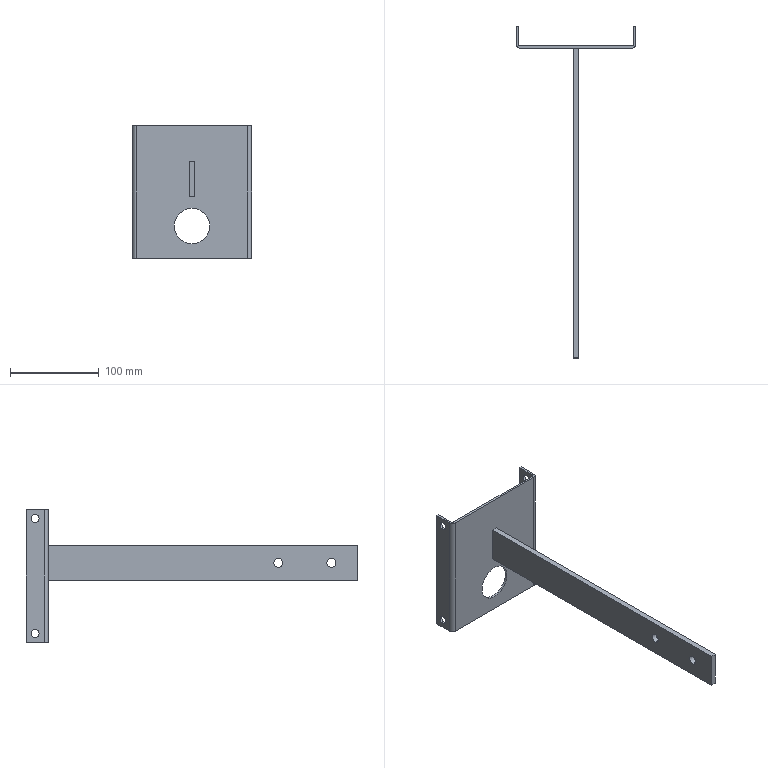Component | SolidWorks | SeedBoxBracket-1 | 1 solid | 33 faces | box 135 x 375 x 150 mm | volume 145734 mm3 | cylinder 18 | plane 15 | commonest cylinder face diameters 9 x10 10 x4 40 x2 4 x2
build123d program:
from build123d import *

# Parameters (mm, degrees)
EXTRUDE_THIN1_DEPTH = 75
SKETCH2_R           = 4.5
CUT_EXTRUDE1_DEPTH  = 157.445
SKETCH3_W           = 6
SKETCH3_H           = 40
BOSS_EXTRUDE1_DEPTH = 350
SKETCH4_R           = 5
CUT_EXTRUDE2_DEPTH  = 400
SKETCH5_R           = 20
CUT_EXTRUDE3_DEPTH  = 10


with BuildPart() as part:
    # Sketch1 → Extrude-Thin1 (new, symmetric)
    with BuildSketch(Plane.XY):
        with BuildLine():
            Line((-67.5, 25), (-67.5, 4.5))
            ThreePointArc((-67.5, 4.5), (-66.182, 1.318), (-63, 0))
            Line((-63, 0), (63, 0))
            ThreePointArc((63, 0), (66.182, 1.318), (67.5, 4.5))
            Line((67.5, 4.5), (67.5, 25))
            Line((67.5, 25), (65, 25))
            Line((65, 25), (65, 4.5))
            ThreePointArc((65, 4.5), (64.414, 3.086), (63, 2.5))
            Line((63, 2.5), (-63, 2.5))
            ThreePointArc((-63, 2.5), (-64.414, 3.086), (-65, 4.5))
            Line((-65, 4.5), (-65, 25))
            Line((-65, 25), (-67.5, 25))
        make_face()
    extrude(amount=EXTRUDE_THIN1_DEPTH, both=True)

    # Sketch2 → Cut-Extrude1 (cut, through all)
    with BuildSketch(Plane.ZY.offset(67.5)):
        with Locations(Location((-65, 14.75, 0), (0, 0, 270))):
            Circle(SKETCH2_R)
        with Locations(Location((65, 14.75, 0), (0, 0, 270))):
            Circle(SKETCH2_R)
    extrude(amount=-CUT_EXTRUDE1_DEPTH, mode=Mode.SUBTRACT)

    # Sketch3 → Boss-Extrude1 (add)
    with BuildSketch(Plane.XZ):
        with Locations((0, -15)):
            Rectangle(SKETCH3_W, SKETCH3_H)
    extrude(amount=BOSS_EXTRUDE1_DEPTH)

    # Sketch4 → Cut-Extrude2 (cut)
    with BuildSketch(Plane.ZY.offset(3)):
        with Locations((-15, -320)):
            Circle(SKETCH4_R)
        with Locations((-15, -260)):
            Circle(SKETCH4_R)
    extrude(amount=-CUT_EXTRUDE2_DEPTH, mode=Mode.SUBTRACT)

    # Sketch5 → Cut-Extrude3 (cut)
    with BuildSketch(Plane(origin=(0, 2.5, 0), x_dir=(1, 0, 0), z_dir=(0, 1, 0))):
        with Locations(Location((0, -38.536, 0), (0, 0, 270))):
            Circle(SKETCH5_R)
    extrude(amount=-CUT_EXTRUDE3_DEPTH, mode=Mode.SUBTRACT)


solid = part.part

# Placed as in the assembly
solid = solid.moved(Location((-5.5, 260, -327.5), (-180, 0, 180)))
STEP:
#1=CARTESIAN_POINT('',(-0.2165,10.236,-13.623));
#2=VERTEX_POINT('',#1);
#3=CARTESIAN_POINT('',(-0.2165,10.236,-15.198));
#4=VERTEX_POINT('',#3);
#5=CARTESIAN_POINT('',(-0.2165,10.236,-14.411));
#6=DIRECTION('',(-0.,1.,0.));
#7=DIRECTION('',(-0.,0.,-1.));
#8=AXIS2_PLACEMENT_3D('',#5,#6,#7);
#9=CIRCLE('',#8,0.7874);
#10=EDGE_CURVE('',#2,#4,#9,.T.);
#11=ORIENTED_EDGE('',*,*,#10,.F.);
#12=CARTESIAN_POINT('',(-0.2165,10.335,-13.623));
#13=VERTEX_POINT('',#12);
#14=CARTESIAN_POINT('',(-0.2165,9.941,-13.623));
#15=DIRECTION('',(-0.,1.,0.));
#16=VECTOR('',#15,39.37);
#17=LINE('',#14,#16);
#18=EDGE_CURVE('',#2,#13,#17,.T.);
#19=ORIENTED_EDGE('',*,*,#18,.T.);
#20=CARTESIAN_POINT('',(-0.2165,10.335,-15.198));
#21=VERTEX_POINT('',#20);
#22=CARTESIAN_POINT('',(-0.2165,10.335,-14.411));
#23=DIRECTION('',(-0.,1.,0.));
#24=DIRECTION('',(-0.,0.,-1.));
#25=AXIS2_PLACEMENT_3D('',#22,#23,#24);
#26=CIRCLE('',#25,0.7874);
#27=EDGE_CURVE('',#13,#21,#26,.T.);
#28=ORIENTED_EDGE('',*,*,#27,.T.);
#29=CARTESIAN_POINT('',(-0.2165,9.941,-15.198));
#30=DIRECTION('',(-0.,1.,0.));
#31=VECTOR('',#30,39.37);
#32=LINE('',#29,#31);
#33=EDGE_CURVE('',#4,#21,#32,.T.);
#34=ORIENTED_EDGE('',*,*,#33,.F.);
#35=EDGE_LOOP('',(#11,#19,#28,#34));
#36=FACE_OUTER_BOUND('',#35,.T.);
#37=CARTESIAN_POINT('',(-0.2165,9.941,-14.411));
#38=DIRECTION('',(-0.,1.,0.));
#39=DIRECTION('',(-0.,0.,-1.));
#40=AXIS2_PLACEMENT_3D('',#37,#38,#39);
#41=CYLINDRICAL_SURFACE('',#40,0.7874);
#42=ADVANCED_FACE('',(#36),#41,.F.);
#43=CARTESIAN_POINT('',(-0.3346,0.,-12.106));
#44=VERTEX_POINT('',#43);
#45=CARTESIAN_POINT('',(-0.3346,0.,-12.5));
#46=VERTEX_POINT('',#45);
#47=CARTESIAN_POINT('',(-0.3346,0.,-12.303));
#48=DIRECTION('',(1.,0.,-0.));
#49=DIRECTION('',(0.,0.,-1.));
#50=AXIS2_PLACEMENT_3D('',#47,#48,#49);
#51=CIRCLE('',#50,0.1969);
#52=EDGE_CURVE('',#44,#46,#51,.T.);
#53=ORIENTED_EDGE('',*,*,#52,.F.);
#54=CARTESIAN_POINT('',(-0.09843,0.,-12.106));
#55=VERTEX_POINT('',#54);
#56=CARTESIAN_POINT('',(-15.846,0.,-12.106));
#57=DIRECTION('',(1.,0.,-0.));
#58=VECTOR('',#57,39.37);
#59=LINE('',#56,#58);
#60=EDGE_CURVE('',#44,#55,#59,.T.);
#61=ORIENTED_EDGE('',*,*,#60,.T.);
#62=CARTESIAN_POINT('',(-0.09843,0.,-12.5));
#63=VERTEX_POINT('',#62);
#64=CARTESIAN_POINT('',(-0.09843,0.,-12.303));
#65=DIRECTION('',(1.,0.,-0.));
#66=DIRECTION('',(-0.,0.,-1.));
#67=AXIS2_PLACEMENT_3D('',#64,#65,#66);
#68=CIRCLE('',#67,0.1969);
#69=EDGE_CURVE('',#55,#63,#68,.T.);
#70=ORIENTED_EDGE('',*,*,#69,.T.);
#71=CARTESIAN_POINT('',(-15.846,0.,-12.5));
#72=DIRECTION('',(1.,0.,-0.));
#73=VECTOR('',#72,39.37);
#74=LINE('',#71,#73);
#75=EDGE_CURVE('',#46,#63,#74,.T.);
#76=ORIENTED_EDGE('',*,*,#75,.F.);
#77=EDGE_LOOP('',(#53,#61,#70,#76));
#78=FACE_OUTER_BOUND('',#77,.T.);
#79=CARTESIAN_POINT('',(-15.846,0.,-12.303));
#80=DIRECTION('',(1.,0.,-0.));
#81=DIRECTION('',(0.,0.,-1.));
#82=AXIS2_PLACEMENT_3D('',#79,#80,#81);
#83=CYLINDRICAL_SURFACE('',#82,0.1969);
#84=ADVANCED_FACE('',(#78),#83,.F.);
#85=CARTESIAN_POINT('',(-0.3346,-2.362,-12.106));
#86=VERTEX_POINT('',#85);
#87=CARTESIAN_POINT('',(-0.3346,-2.362,-12.5));
#88=VERTEX_POINT('',#87);
#89=CARTESIAN_POINT('',(-0.3346,-2.362,-12.303));
#90=DIRECTION('',(1.,0.,-0.));
#91=DIRECTION('',(0.,0.,-1.));
#92=AXIS2_PLACEMENT_3D('',#89,#90,#91);
#93=CIRCLE('',#92,0.1969);
#94=EDGE_CURVE('',#86,#88,#93,.T.);
#95=ORIENTED_EDGE('',*,*,#94,.F.);
#96=CARTESIAN_POINT('',(-0.09843,-2.362,-12.106));
#97=VERTEX_POINT('',#96);
#98=CARTESIAN_POINT('',(-15.846,-2.362,-12.106));
#99=DIRECTION('',(1.,0.,-0.));
#100=VECTOR('',#99,39.37);
#101=LINE('',#98,#100);
#102=EDGE_CURVE('',#86,#97,#101,.T.);
#103=ORIENTED_EDGE('',*,*,#102,.T.);
#104=CARTESIAN_POINT('',(-0.09843,-2.362,-12.5));
#105=VERTEX_POINT('',#104);
#106=CARTESIAN_POINT('',(-0.09843,-2.362,-12.303));
#107=DIRECTION('',(1.,0.,-0.));
#108=DIRECTION('',(-0.,0.,-1.));
#109=AXIS2_PLACEMENT_3D('',#106,#107,#108);
#110=CIRCLE('',#109,0.1969);
#111=EDGE_CURVE('',#97,#105,#110,.T.);
#112=ORIENTED_EDGE('',*,*,#111,.T.);
#113=CARTESIAN_POINT('',(-15.846,-2.362,-12.5));
#114=DIRECTION('',(1.,0.,-0.));
#115=VECTOR('',#114,39.37);
#116=LINE('',#113,#115);
#117=EDGE_CURVE('',#88,#105,#116,.T.);
#118=ORIENTED_EDGE('',*,*,#117,.F.);
#119=EDGE_LOOP('',(#95,#103,#112,#118));
#120=FACE_OUTER_BOUND('',#119,.T.);
#121=CARTESIAN_POINT('',(-15.846,-2.362,-12.303));
#122=DIRECTION('',(1.,0.,-0.));
#123=DIRECTION('',(0.,0.,-1.));
#124=AXIS2_PLACEMENT_3D('',#121,#122,#123);
#125=CYLINDRICAL_SURFACE('',#124,0.1969);
#126=ADVANCED_FACE('',(#120),#125,.F.);
#127=CARTESIAN_POINT('',(-2.874,10.994,-15.453));
#128=VERTEX_POINT('',#127);
#129=CARTESIAN_POINT('',(-2.874,10.64,-15.453));
#130=VERTEX_POINT('',#129);
#131=CARTESIAN_POINT('',(-2.874,10.817,-15.453));
#132=DIRECTION('',(1.,-0.,-0.));
#133=DIRECTION('',(0.,-1.,0.));
#134=AXIS2_PLACEMENT_3D('',#131,#132,#133);
#135=CIRCLE('',#134,0.1772);
#136=EDGE_CURVE('',#128,#130,#135,.T.);
#137=ORIENTED_EDGE('',*,*,#136,.F.);
#138=CARTESIAN_POINT('',(-2.776,10.994,-15.453));
#139=VERTEX_POINT('',#138);
#140=CARTESIAN_POINT('',(-2.874,10.994,-15.453));
#141=DIRECTION('',(1.,-0.,-0.));
#142=VECTOR('',#141,39.37);
#143=LINE('',#140,#142);
#144=EDGE_CURVE('',#128,#139,#143,.T.);
#145=ORIENTED_EDGE('',*,*,#144,.T.);
#146=CARTESIAN_POINT('',(-2.776,10.64,-15.453));
#147=VERTEX_POINT('',#146);
#148=CARTESIAN_POINT('',(-2.776,10.817,-15.453));
#149=DIRECTION('',(1.,0.,-0.));
#150=DIRECTION('',(0.,0.,-1.));
#151=AXIS2_PLACEMENT_3D('',#148,#149,#150);
#152=CIRCLE('',#151,0.1772);
#153=EDGE_CURVE('',#139,#147,#152,.T.);
#154=ORIENTED_EDGE('',*,*,#153,.T.);
#155=CARTESIAN_POINT('',(-2.874,10.64,-15.453));
#156=DIRECTION('',(1.,-0.,-0.));
#157=VECTOR('',#156,39.37);
#158=LINE('',#155,#157);
#159=EDGE_CURVE('',#130,#147,#158,.T.);
#160=ORIENTED_EDGE('',*,*,#159,.F.);
#161=EDGE_LOOP('',(#137,#145,#154,#160));
#162=FACE_OUTER_BOUND('',#161,.T.);
#163=CARTESIAN_POINT('',(-2.874,10.817,-15.453));
#164=DIRECTION('',(1.,-0.,-0.));
#165=DIRECTION('',(0.,-1.,0.));
#166=AXIS2_PLACEMENT_3D('',#163,#164,#165);
#167=CYLINDRICAL_SURFACE('',#166,0.1772);
#168=ADVANCED_FACE('',(#162),#167,.F.);
#169=CARTESIAN_POINT('',(2.343,10.64,-15.453));
#170=VERTEX_POINT('',#169);
#171=CARTESIAN_POINT('',(2.343,10.994,-15.453));
#172=VERTEX_POINT('',#171);
#173=CARTESIAN_POINT('',(2.343,10.817,-15.453));
#174=DIRECTION('',(-1.,-0.,0.));
#175=DIRECTION('',(0.,0.,1.));
#176=AXIS2_PLACEMENT_3D('',#173,#174,#175);
#177=CIRCLE('',#176,0.1772);
#178=EDGE_CURVE('',#170,#172,#177,.T.);
#179=ORIENTED_EDGE('',*,*,#178,.T.);
#180=CARTESIAN_POINT('',(2.441,10.994,-15.453));
#181=VERTEX_POINT('',#180);
#182=CARTESIAN_POINT('',(-2.874,10.994,-15.453));
#183=DIRECTION('',(1.,-0.,-0.));
#184=VECTOR('',#183,39.37);
#185=LINE('',#182,#184);
#186=EDGE_CURVE('',#172,#181,#185,.T.);
#187=ORIENTED_EDGE('',*,*,#186,.T.);
#188=CARTESIAN_POINT('',(2.441,10.64,-15.453));
#189=VERTEX_POINT('',#188);
#190=CARTESIAN_POINT('',(2.441,10.817,-15.453));
#191=DIRECTION('',(1.,-0.,-0.));
#192=DIRECTION('',(0.,-1.,0.));
#193=AXIS2_PLACEMENT_3D('',#190,#191,#192);
#194=CIRCLE('',#193,0.1772);
#195=EDGE_CURVE('',#181,#189,#194,.T.);
#196=ORIENTED_EDGE('',*,*,#195,.T.);
#197=CARTESIAN_POINT('',(-2.874,10.64,-15.453));
#198=DIRECTION('',(1.,-0.,-0.));
#199=VECTOR('',#198,39.37);
#200=LINE('',#197,#199);
#201=EDGE_CURVE('',#170,#189,#200,.T.);
#202=ORIENTED_EDGE('',*,*,#201,.F.);
#203=EDGE_LOOP('',(#179,#187,#196,#202));
#204=FACE_OUTER_BOUND('',#203,.T.);
#205=CARTESIAN_POINT('',(-2.874,10.817,-15.453));
#206=DIRECTION('',(1.,-0.,-0.));
#207=DIRECTION('',(0.,-1.,0.));
#208=AXIS2_PLACEMENT_3D('',#205,#206,#207);
#209=CYLINDRICAL_SURFACE('',#208,0.1772);
#210=ADVANCED_FACE('',(#204),#209,.F.);
#211=CARTESIAN_POINT('',(-2.874,10.994,-10.335));
#212=VERTEX_POINT('',#211);
#213=CARTESIAN_POINT('',(-2.874,10.64,-10.335));
#214=VERTEX_POINT('',#213);
#215=CARTESIAN_POINT('',(-2.874,10.817,-10.335));
#216=DIRECTION('',(1.,-0.,-0.));
#217=DIRECTION('',(0.,-1.,0.));
#218=AXIS2_PLACEMENT_3D('',#215,#216,#217);
#219=CIRCLE('',#218,0.1772);
#220=EDGE_CURVE('',#212,#214,#219,.T.);
#221=ORIENTED_EDGE('',*,*,#220,.F.);
#222=CARTESIAN_POINT('',(-2.776,10.994,-10.335));
#223=VERTEX_POINT('',#222);
#224=CARTESIAN_POINT('',(-2.874,10.994,-10.335));
#225=DIRECTION('',(1.,-0.,-0.));
#226=VECTOR('',#225,39.37);
#227=LINE('',#224,#226);
#228=EDGE_CURVE('',#212,#223,#227,.T.);
#229=ORIENTED_EDGE('',*,*,#228,.T.);
#230=CARTESIAN_POINT('',(-2.776,10.64,-10.335));
#231=VERTEX_POINT('',#230);
#232=CARTESIAN_POINT('',(-2.776,10.817,-10.335));
#233=DIRECTION('',(1.,0.,-0.));
#234=DIRECTION('',(0.,0.,-1.));
#235=AXIS2_PLACEMENT_3D('',#232,#233,#234);
#236=CIRCLE('',#235,0.1772);
#237=EDGE_CURVE('',#223,#231,#236,.T.);
#238=ORIENTED_EDGE('',*,*,#237,.T.);
#239=CARTESIAN_POINT('',(-2.874,10.64,-10.335));
#240=DIRECTION('',(1.,-0.,-0.));
#241=VECTOR('',#240,39.37);
#242=LINE('',#239,#241);
#243=EDGE_CURVE('',#214,#231,#242,.T.);
#244=ORIENTED_EDGE('',*,*,#243,.F.);
#245=EDGE_LOOP('',(#221,#229,#238,#244));
#246=FACE_OUTER_BOUND('',#245,.T.);
#247=CARTESIAN_POINT('',(-2.874,10.817,-10.335));
#248=DIRECTION('',(1.,-0.,-0.));
#249=DIRECTION('',(0.,-1.,0.));
#250=AXIS2_PLACEMENT_3D('',#247,#248,#249);
#251=CYLINDRICAL_SURFACE('',#250,0.1772);
#252=ADVANCED_FACE('',(#246),#251,.F.);
#253=CARTESIAN_POINT('',(2.343,10.64,-10.335));
#254=VERTEX_POINT('',#253);
#255=CARTESIAN_POINT('',(2.343,10.994,-10.335));
#256=VERTEX_POINT('',#255);
#257=CARTESIAN_POINT('',(2.343,10.817,-10.335));
#258=DIRECTION('',(-1.,-0.,0.));
#259=DIRECTION('',(0.,0.,1.));
#260=AXIS2_PLACEMENT_3D('',#257,#258,#259);
#261=CIRCLE('',#260,0.1772);
#262=EDGE_CURVE('',#254,#256,#261,.T.);
#263=ORIENTED_EDGE('',*,*,#262,.T.);
#264=CARTESIAN_POINT('',(2.441,10.994,-10.335));
#265=VERTEX_POINT('',#264);
#266=CARTESIAN_POINT('',(-2.874,10.994,-10.335));
#267=DIRECTION('',(1.,-0.,-0.));
#268=VECTOR('',#267,39.37);
#269=LINE('',#266,#268);
#270=EDGE_CURVE('',#256,#265,#269,.T.);
#271=ORIENTED_EDGE('',*,*,#270,.T.);
#272=CARTESIAN_POINT('',(2.441,10.64,-10.335));
#273=VERTEX_POINT('',#272);
#274=CARTESIAN_POINT('',(2.441,10.817,-10.335));
#275=DIRECTION('',(1.,-0.,-0.));
#276=DIRECTION('',(0.,-1.,0.));
#277=AXIS2_PLACEMENT_3D('',#274,#275,#276);
#278=CIRCLE('',#277,0.1772);
#279=EDGE_CURVE('',#265,#273,#278,.T.);
#280=ORIENTED_EDGE('',*,*,#279,.T.);
#281=CARTESIAN_POINT('',(-2.874,10.64,-10.335));
#282=DIRECTION('',(1.,-0.,-0.));
#283=VECTOR('',#282,39.37);
#284=LINE('',#281,#283);
#285=EDGE_CURVE('',#254,#273,#284,.T.);
#286=ORIENTED_EDGE('',*,*,#285,.F.);
#287=EDGE_LOOP('',(#263,#271,#280,#286));
#288=FACE_OUTER_BOUND('',#287,.T.);
#289=CARTESIAN_POINT('',(-2.874,10.817,-10.335));
#290=DIRECTION('',(1.,-0.,-0.));
#291=DIRECTION('',(0.,-1.,0.));
#292=AXIS2_PLACEMENT_3D('',#289,#290,#291);
#293=CYLINDRICAL_SURFACE('',#292,0.1772);
#294=ADVANCED_FACE('',(#288),#293,.F.);
#295=CARTESIAN_POINT('',(-0.2165,10.236,-14.411));
#296=DIRECTION('',(-0.,1.,0.));
#297=DIRECTION('',(-0.,0.,-1.));
#298=AXIS2_PLACEMENT_3D('',#295,#296,#297);
#299=CIRCLE('',#298,0.7874);
#300=EDGE_CURVE('',#4,#2,#299,.T.);
#301=ORIENTED_EDGE('',*,*,#300,.T.);
#302=ORIENTED_EDGE('',*,*,#10,.T.);
#303=EDGE_LOOP('',(#301,#302));
#304=FACE_BOUND('',#303,.T.);
#305=CARTESIAN_POINT('',(2.264,10.236,-9.941));
#306=VERTEX_POINT('',#305);
#307=CARTESIAN_POINT('',(-2.697,10.236,-9.941));
#308=VERTEX_POINT('',#307);
#309=CARTESIAN_POINT('',(2.264,10.236,-9.941));
#310=DIRECTION('',(-1.,-0.,0.));
#311=VECTOR('',#310,39.37);
#312=LINE('',#309,#311);
#313=EDGE_CURVE('',#306,#308,#312,.T.);
#314=ORIENTED_EDGE('',*,*,#313,.T.);
#315=CARTESIAN_POINT('',(-2.697,10.236,-15.846));
#316=VERTEX_POINT('',#315);
#317=CARTESIAN_POINT('',(-2.697,10.236,-15.846));
#318=DIRECTION('',(0.,0.,1.));
#319=VECTOR('',#318,39.37);
#320=LINE('',#317,#319);
#321=EDGE_CURVE('',#316,#308,#320,.T.);
#322=ORIENTED_EDGE('',*,*,#321,.F.);
#323=CARTESIAN_POINT('',(2.264,10.236,-15.846));
#324=VERTEX_POINT('',#323);
#325=CARTESIAN_POINT('',(2.264,10.236,-15.846));
#326=DIRECTION('',(-1.,-0.,0.));
#327=VECTOR('',#326,39.37);
#328=LINE('',#325,#327);
#329=EDGE_CURVE('',#324,#316,#328,.T.);
#330=ORIENTED_EDGE('',*,*,#329,.F.);
#331=CARTESIAN_POINT('',(2.264,10.236,-15.846));
#332=DIRECTION('',(0.,0.,1.));
#333=VECTOR('',#332,39.37);
#334=LINE('',#331,#333);
#335=EDGE_CURVE('',#324,#306,#334,.T.);
#336=ORIENTED_EDGE('',*,*,#335,.T.);
#337=EDGE_LOOP('',(#314,#322,#330,#336));
#338=FACE_OUTER_BOUND('',#337,.T.);
#339=CARTESIAN_POINT('',(-0.3346,10.236,-11.516));
#340=VERTEX_POINT('',#339);
#341=CARTESIAN_POINT('',(-0.3346,10.236,-13.091));
#342=VERTEX_POINT('',#341);
#343=CARTESIAN_POINT('',(-0.3346,10.236,-11.516));
#344=DIRECTION('',(-0.,0.,-1.));
#345=VECTOR('',#344,39.37);
#346=LINE('',#343,#345);
#347=EDGE_CURVE('',#340,#342,#346,.T.);
#348=ORIENTED_EDGE('',*,*,#347,.F.);
#349=CARTESIAN_POINT('',(-0.09843,10.236,-11.516));
#350=VERTEX_POINT('',#349);
#351=CARTESIAN_POINT('',(-0.09843,10.236,-11.516));
#352=DIRECTION('',(-1.,-0.,0.));
#353=VECTOR('',#352,39.37);
#354=LINE('',#351,#353);
#355=EDGE_CURVE('',#350,#340,#354,.T.);
#356=ORIENTED_EDGE('',*,*,#355,.F.);
#357=CARTESIAN_POINT('',(-0.09843,10.236,-13.091));
#358=VERTEX_POINT('',#357);
#359=CARTESIAN_POINT('',(-0.09843,10.236,-11.516));
#360=DIRECTION('',(0.,0.,1.));
#361=VECTOR('',#360,39.37);
#362=LINE('',#359,#361);
#363=EDGE_CURVE('',#358,#350,#362,.T.);
#364=ORIENTED_EDGE('',*,*,#363,.F.);
#365=CARTESIAN_POINT('',(-0.09843,10.236,-13.091));
#366=DIRECTION('',(1.,0.,-0.));
#367=VECTOR('',#366,39.37);
#368=LINE('',#365,#367);
#369=EDGE_CURVE('',#342,#358,#368,.T.);
#370=ORIENTED_EDGE('',*,*,#369,.F.);
#371=EDGE_LOOP('',(#348,#356,#364,#370));
#372=FACE_BOUND('',#371,.T.);
#373=CARTESIAN_POINT('',(2.264,10.236,-15.846));
#374=DIRECTION('',(-0.,1.,0.));
#375=DIRECTION('',(-0.,0.,-1.));
#376=AXIS2_PLACEMENT_3D('',#373,#374,#375);
#377=PLANE('',#376);
#378=ADVANCED_FACE('',(#304,#338,#372),#377,.F.);
#379=CARTESIAN_POINT('',(-2.874,10.817,-15.453));
#380=DIRECTION('',(1.,-0.,-0.));
#381=DIRECTION('',(0.,-1.,0.));
#382=AXIS2_PLACEMENT_3D('',#379,#380,#381);
#383=CIRCLE('',#382,0.1772);
#384=EDGE_CURVE('',#130,#128,#383,.T.);
#385=ORIENTED_EDGE('',*,*,#384,.T.);
#386=ORIENTED_EDGE('',*,*,#136,.T.);
#387=EDGE_LOOP('',(#385,#386));
#388=FACE_BOUND('',#387,.T.);
#389=CARTESIAN_POINT('',(-2.874,10.817,-10.335));
#390=DIRECTION('',(1.,-0.,-0.));
#391=DIRECTION('',(0.,-1.,0.));
#392=AXIS2_PLACEMENT_3D('',#389,#390,#391);
#393=CIRCLE('',#392,0.1772);
#394=EDGE_CURVE('',#214,#212,#393,.T.);
#395=ORIENTED_EDGE('',*,*,#394,.T.);
#396=ORIENTED_EDGE('',*,*,#220,.T.);
#397=EDGE_LOOP('',(#395,#396));
#398=FACE_BOUND('',#397,.T.);
#399=CARTESIAN_POINT('',(-2.874,10.413,-9.941));
#400=VERTEX_POINT('',#399);
#401=CARTESIAN_POINT('',(-2.874,11.22,-9.941));
#402=VERTEX_POINT('',#401);
#403=CARTESIAN_POINT('',(-2.874,10.413,-9.941));
#404=DIRECTION('',(-0.,1.,0.));
#405=VECTOR('',#404,39.37);
#406=LINE('',#403,#405);
#407=EDGE_CURVE('',#400,#402,#406,.T.);
#408=ORIENTED_EDGE('',*,*,#407,.T.);
#409=CARTESIAN_POINT('',(-2.874,11.22,-15.846));
#410=VERTEX_POINT('',#409);
#411=CARTESIAN_POINT('',(-2.874,11.22,-15.846));
#412=DIRECTION('',(0.,0.,1.));
#413=VECTOR('',#412,39.37);
#414=LINE('',#411,#413);
#415=EDGE_CURVE('',#410,#402,#414,.T.);
#416=ORIENTED_EDGE('',*,*,#415,.F.);
#417=CARTESIAN_POINT('',(-2.874,10.413,-15.846));
#418=VERTEX_POINT('',#417);
#419=CARTESIAN_POINT('',(-2.874,10.413,-15.846));
#420=DIRECTION('',(-0.,1.,0.));
#421=VECTOR('',#420,39.37);
#422=LINE('',#419,#421);
#423=EDGE_CURVE('',#418,#410,#422,.T.);
#424=ORIENTED_EDGE('',*,*,#423,.F.);
#425=CARTESIAN_POINT('',(-2.874,10.413,-15.846));
#426=DIRECTION('',(0.,0.,1.));
#427=VECTOR('',#426,39.37);
#428=LINE('',#425,#427);
#429=EDGE_CURVE('',#418,#400,#428,.T.);
#430=ORIENTED_EDGE('',*,*,#429,.T.);
#431=EDGE_LOOP('',(#408,#416,#424,#430));
#432=FACE_OUTER_BOUND('',#431,.T.);
#433=CARTESIAN_POINT('',(-2.874,10.413,-15.846));
#434=DIRECTION('',(1.,0.,-0.));
#435=DIRECTION('',(-0.,0.,-1.));
#436=AXIS2_PLACEMENT_3D('',#433,#434,#435);
#437=PLANE('',#436);
#438=ADVANCED_FACE('',(#388,#398,#432),#437,.F.);
#439=CARTESIAN_POINT('',(-2.776,11.22,-9.941));
#440=VERTEX_POINT('',#439);
#441=CARTESIAN_POINT('',(-2.776,11.22,-9.941));
#442=DIRECTION('',(-1.,-0.,0.));
#443=VECTOR('',#442,39.37);
#444=LINE('',#441,#443);
#445=EDGE_CURVE('',#440,#402,#444,.T.);
#446=ORIENTED_EDGE('',*,*,#445,.F.);
#447=CARTESIAN_POINT('',(-2.776,11.22,-15.846));
#448=VERTEX_POINT('',#447);
#449=CARTESIAN_POINT('',(-2.776,11.22,-15.846));
#450=DIRECTION('',(0.,0.,1.));
#451=VECTOR('',#450,39.37);
#452=LINE('',#449,#451);
#453=EDGE_CURVE('',#448,#440,#452,.T.);
#454=ORIENTED_EDGE('',*,*,#453,.F.);
#455=CARTESIAN_POINT('',(-2.776,11.22,-15.846));
#456=DIRECTION('',(-1.,-0.,0.));
#457=VECTOR('',#456,39.37);
#458=LINE('',#455,#457);
#459=EDGE_CURVE('',#448,#410,#458,.T.);
#460=ORIENTED_EDGE('',*,*,#459,.T.);
#461=ORIENTED_EDGE('',*,*,#415,.T.);
#462=EDGE_LOOP('',(#446,#454,#460,#461));
#463=FACE_OUTER_BOUND('',#462,.T.);
#464=CARTESIAN_POINT('',(-2.776,11.22,-15.846));
#465=DIRECTION('',(-0.,1.,0.));
#466=DIRECTION('',(-0.,0.,-1.));
#467=AXIS2_PLACEMENT_3D('',#464,#465,#466);
#468=PLANE('',#467);
#469=ADVANCED_FACE('',(#463),#468,.T.);
#470=CARTESIAN_POINT('',(-2.776,10.817,-15.453));
#471=DIRECTION('',(1.,0.,-0.));
#472=DIRECTION('',(0.,0.,-1.));
#473=AXIS2_PLACEMENT_3D('',#470,#471,#472);
#474=CIRCLE('',#473,0.1772);
#475=EDGE_CURVE('',#147,#139,#474,.T.);
#476=ORIENTED_EDGE('',*,*,#475,.F.);
#477=ORIENTED_EDGE('',*,*,#153,.F.);
#478=EDGE_LOOP('',(#476,#477));
#479=FACE_BOUND('',#478,.T.);
#480=CARTESIAN_POINT('',(-2.776,10.817,-10.335));
#481=DIRECTION('',(1.,0.,-0.));
#482=DIRECTION('',(0.,0.,-1.));
#483=AXIS2_PLACEMENT_3D('',#480,#481,#482);
#484=CIRCLE('',#483,0.1772);
#485=EDGE_CURVE('',#231,#223,#484,.T.);
#486=ORIENTED_EDGE('',*,*,#485,.F.);
#487=ORIENTED_EDGE('',*,*,#237,.F.);
#488=EDGE_LOOP('',(#486,#487));
#489=FACE_BOUND('',#488,.T.);
#490=CARTESIAN_POINT('',(-2.776,10.413,-9.941));
#491=VERTEX_POINT('',#490);
#492=CARTESIAN_POINT('',(-2.776,10.413,-9.941));
#493=DIRECTION('',(-0.,1.,0.));
#494=VECTOR('',#493,39.37);
#495=LINE('',#492,#494);
#496=EDGE_CURVE('',#491,#440,#495,.T.);
#497=ORIENTED_EDGE('',*,*,#496,.F.);
#498=CARTESIAN_POINT('',(-2.776,10.413,-15.846));
#499=VERTEX_POINT('',#498);
#500=CARTESIAN_POINT('',(-2.776,10.413,-15.846));
#501=DIRECTION('',(0.,0.,1.));
#502=VECTOR('',#501,39.37);
#503=LINE('',#500,#502);
#504=EDGE_CURVE('',#499,#491,#503,.T.);
#505=ORIENTED_EDGE('',*,*,#504,.F.);
#506=CARTESIAN_POINT('',(-2.776,10.413,-15.846));
#507=DIRECTION('',(-0.,1.,0.));
#508=VECTOR('',#507,39.37);
#509=LINE('',#506,#508);
#510=EDGE_CURVE('',#499,#448,#509,.T.);
#511=ORIENTED_EDGE('',*,*,#510,.T.);
#512=ORIENTED_EDGE('',*,*,#453,.T.);
#513=EDGE_LOOP('',(#497,#505,#511,#512));
#514=FACE_OUTER_BOUND('',#513,.T.);
#515=CARTESIAN_POINT('',(-2.776,10.413,-15.846));
#516=DIRECTION('',(1.,0.,-0.));
#517=DIRECTION('',(-0.,0.,-1.));
#518=AXIS2_PLACEMENT_3D('',#515,#516,#517);
#519=PLANE('',#518);
#520=ADVANCED_FACE('',(#479,#489,#514),#519,.T.);
#521=CARTESIAN_POINT('',(-2.697,10.335,-9.941));
#522=VERTEX_POINT('',#521);
#523=CARTESIAN_POINT('',(-2.697,10.413,-9.941));
#524=DIRECTION('',(-0.,0.,-1.));
#525=DIRECTION('',(-1.,0.,0.));
#526=AXIS2_PLACEMENT_3D('',#523,#524,#525);
#527=CIRCLE('',#526,0.07874);
#528=EDGE_CURVE('',#522,#491,#527,.T.);
#529=ORIENTED_EDGE('',*,*,#528,.F.);
#530=CARTESIAN_POINT('',(-2.697,10.335,-15.846));
#531=VERTEX_POINT('',#530);
#532=CARTESIAN_POINT('',(-2.697,10.335,-15.846));
#533=DIRECTION('',(0.,0.,1.));
#534=VECTOR('',#533,39.37);
#535=LINE('',#532,#534);
#536=EDGE_CURVE('',#531,#522,#535,.T.);
#537=ORIENTED_EDGE('',*,*,#536,.F.);
#538=CARTESIAN_POINT('',(-2.697,10.413,-15.846));
#539=DIRECTION('',(-0.,0.,-1.));
#540=DIRECTION('',(-1.,0.,0.));
#541=AXIS2_PLACEMENT_3D('',#538,#539,#540);
#542=CIRCLE('',#541,0.07874);
#543=EDGE_CURVE('',#531,#499,#542,.T.);
#544=ORIENTED_EDGE('',*,*,#543,.T.);
#545=ORIENTED_EDGE('',*,*,#504,.T.);
#546=EDGE_LOOP('',(#529,#537,#544,#545));
#547=FACE_OUTER_BOUND('',#546,.T.);
#548=CARTESIAN_POINT('',(-2.697,10.413,-15.846));
#549=DIRECTION('',(0.,0.,1.));
#550=DIRECTION('',(1.,0.,0.));
#551=AXIS2_PLACEMENT_3D('',#548,#549,#550);
#552=CYLINDRICAL_SURFACE('',#551,0.07874);
#553=ADVANCED_FACE('',(#547),#552,.F.);
#554=CARTESIAN_POINT('',(-0.2165,10.335,-14.411));
#555=DIRECTION('',(-0.,1.,0.));
#556=DIRECTION('',(-0.,0.,-1.));
#557=AXIS2_PLACEMENT_3D('',#554,#555,#556);
#558=CIRCLE('',#557,0.7874);
#559=EDGE_CURVE('',#21,#13,#558,.T.);
#560=ORIENTED_EDGE('',*,*,#559,.F.);
#561=ORIENTED_EDGE('',*,*,#27,.F.);
#562=EDGE_LOOP('',(#560,#561));
#563=FACE_BOUND('',#562,.T.);
#564=CARTESIAN_POINT('',(2.264,10.335,-9.941));
#565=VERTEX_POINT('',#564);
#566=CARTESIAN_POINT('',(2.264,10.335,-9.941));
#567=DIRECTION('',(-1.,-0.,0.));
#568=VECTOR('',#567,39.37);
#569=LINE('',#566,#568);
#570=EDGE_CURVE('',#565,#522,#569,.T.);
#571=ORIENTED_EDGE('',*,*,#570,.F.);
#572=CARTESIAN_POINT('',(2.264,10.335,-15.846));
#573=VERTEX_POINT('',#572);
#574=CARTESIAN_POINT('',(2.264,10.335,-15.846));
#575=DIRECTION('',(0.,0.,1.));
#576=VECTOR('',#575,39.37);
#577=LINE('',#574,#576);
#578=EDGE_CURVE('',#573,#565,#577,.T.);
#579=ORIENTED_EDGE('',*,*,#578,.F.);
#580=CARTESIAN_POINT('',(2.264,10.335,-15.846));
#581=DIRECTION('',(-1.,-0.,0.));
#582=VECTOR('',#581,39.37);
#583=LINE('',#580,#582);
#584=EDGE_CURVE('',#573,#531,#583,.T.);
#585=ORIENTED_EDGE('',*,*,#584,.T.);
#586=ORIENTED_EDGE('',*,*,#536,.T.);
#587=EDGE_LOOP('',(#571,#579,#585,#586));
#588=FACE_OUTER_BOUND('',#587,.T.);
#589=CARTESIAN_POINT('',(2.264,10.335,-15.846));
#590=DIRECTION('',(-0.,1.,0.));
#591=DIRECTION('',(-0.,0.,-1.));
#592=AXIS2_PLACEMENT_3D('',#589,#590,#591);
#593=PLANE('',#592);
#594=ADVANCED_FACE('',(#563,#588),#593,.T.);
#595=CARTESIAN_POINT('',(2.343,10.413,-9.941));
#596=VERTEX_POINT('',#595);
#597=CARTESIAN_POINT('',(2.264,10.413,-9.941));
#598=DIRECTION('',(-0.,0.,-1.));
#599=DIRECTION('',(-1.,0.,0.));
#600=AXIS2_PLACEMENT_3D('',#597,#598,#599);
#601=CIRCLE('',#600,0.07874);
#602=EDGE_CURVE('',#596,#565,#601,.T.);
#603=ORIENTED_EDGE('',*,*,#602,.F.);
#604=CARTESIAN_POINT('',(2.343,10.413,-15.846));
#605=VERTEX_POINT('',#604);
#606=CARTESIAN_POINT('',(2.343,10.413,-15.846));
#607=DIRECTION('',(0.,0.,1.));
#608=VECTOR('',#607,39.37);
#609=LINE('',#606,#608);
#610=EDGE_CURVE('',#605,#596,#609,.T.);
#611=ORIENTED_EDGE('',*,*,#610,.F.);
#612=CARTESIAN_POINT('',(2.264,10.413,-15.846));
#613=DIRECTION('',(-0.,0.,-1.));
#614=DIRECTION('',(-1.,0.,0.));
#615=AXIS2_PLACEMENT_3D('',#612,#613,#614);
#616=CIRCLE('',#615,0.07874);
#617=EDGE_CURVE('',#605,#573,#616,.T.);
#618=ORIENTED_EDGE('',*,*,#617,.T.);
#619=ORIENTED_EDGE('',*,*,#578,.T.);
#620=EDGE_LOOP('',(#603,#611,#618,#619));
#621=FACE_OUTER_BOUND('',#620,.T.);
#622=CARTESIAN_POINT('',(2.264,10.413,-15.846));
#623=DIRECTION('',(0.,0.,1.));
#624=DIRECTION('',(1.,0.,0.));
#625=AXIS2_PLACEMENT_3D('',#622,#623,#624);
#626=CYLINDRICAL_SURFACE('',#625,0.07874);
#627=ADVANCED_FACE('',(#621),#626,.F.);
#628=ORIENTED_EDGE('',*,*,#178,.F.);
#629=CARTESIAN_POINT('',(2.343,10.817,-15.453));
#630=DIRECTION('',(-1.,-0.,0.));
#631=DIRECTION('',(0.,0.,1.));
#632=AXIS2_PLACEMENT_3D('',#629,#630,#631);
#633=CIRCLE('',#632,0.1772);
#634=EDGE_CURVE('',#172,#170,#633,.T.);
#635=ORIENTED_EDGE('',*,*,#634,.F.);
#636=EDGE_LOOP('',(#628,#635));
#637=FACE_BOUND('',#636,.T.);
#638=ORIENTED_EDGE('',*,*,#262,.F.);
#639=CARTESIAN_POINT('',(2.343,10.817,-10.335));
#640=DIRECTION('',(-1.,-0.,0.));
#641=DIRECTION('',(0.,0.,1.));
#642=AXIS2_PLACEMENT_3D('',#639,#640,#641);
#643=CIRCLE('',#642,0.1772);
#644=EDGE_CURVE('',#256,#254,#643,.T.);
#645=ORIENTED_EDGE('',*,*,#644,.F.);
#646=EDGE_LOOP('',(#638,#645));
#647=FACE_BOUND('',#646,.T.);
#648=CARTESIAN_POINT('',(2.343,11.22,-9.941));
#649=VERTEX_POINT('',#648);
#650=CARTESIAN_POINT('',(2.343,11.22,-9.941));
#651=DIRECTION('',(0.,-1.,0.));
#652=VECTOR('',#651,39.37);
#653=LINE('',#650,#652);
#654=EDGE_CURVE('',#649,#596,#653,.T.);
#655=ORIENTED_EDGE('',*,*,#654,.F.);
#656=CARTESIAN_POINT('',(2.343,11.22,-15.846));
#657=VERTEX_POINT('',#656);
#658=CARTESIAN_POINT('',(2.343,11.22,-15.846));
#659=DIRECTION('',(0.,0.,1.));
#660=VECTOR('',#659,39.37);
#661=LINE('',#658,#660);
#662=EDGE_CURVE('',#657,#649,#661,.T.);
#663=ORIENTED_EDGE('',*,*,#662,.F.);
#664=CARTESIAN_POINT('',(2.343,11.22,-15.846));
#665=DIRECTION('',(0.,-1.,0.));
#666=VECTOR('',#665,39.37);
#667=LINE('',#664,#666);
#668=EDGE_CURVE('',#657,#605,#667,.T.);
#669=ORIENTED_EDGE('',*,*,#668,.T.);
#670=ORIENTED_EDGE('',*,*,#610,.T.);
#671=EDGE_LOOP('',(#655,#663,#669,#670));
#672=FACE_OUTER_BOUND('',#671,.T.);
#673=CARTESIAN_POINT('',(2.343,11.22,-15.846));
#674=DIRECTION('',(-1.,-0.,0.));
#675=DIRECTION('',(0.,0.,1.));
#676=AXIS2_PLACEMENT_3D('',#673,#674,#675);
#677=PLANE('',#676);
#678=ADVANCED_FACE('',(#637,#647,#672),#677,.T.);
#679=CARTESIAN_POINT('',(2.441,11.22,-9.941));
#680=VERTEX_POINT('',#679);
#681=CARTESIAN_POINT('',(2.441,11.22,-9.941));
#682=DIRECTION('',(-1.,-0.,0.));
#683=VECTOR('',#682,39.37);
#684=LINE('',#681,#683);
#685=EDGE_CURVE('',#680,#649,#684,.T.);
#686=ORIENTED_EDGE('',*,*,#685,.F.);
#687=CARTESIAN_POINT('',(2.441,11.22,-15.846));
#688=VERTEX_POINT('',#687);
#689=CARTESIAN_POINT('',(2.441,11.22,-15.846));
#690=DIRECTION('',(0.,0.,1.));
#691=VECTOR('',#690,39.37);
#692=LINE('',#689,#691);
#693=EDGE_CURVE('',#688,#680,#692,.T.);
#694=ORIENTED_EDGE('',*,*,#693,.F.);
#695=CARTESIAN_POINT('',(2.441,11.22,-15.846));
#696=DIRECTION('',(-1.,-0.,0.));
#697=VECTOR('',#696,39.37);
#698=LINE('',#695,#697);
#699=EDGE_CURVE('',#688,#657,#698,.T.);
#700=ORIENTED_EDGE('',*,*,#699,.T.);
#701=ORIENTED_EDGE('',*,*,#662,.T.);
#702=EDGE_LOOP('',(#686,#694,#700,#701));
#703=FACE_OUTER_BOUND('',#702,.T.);
#704=CARTESIAN_POINT('',(2.441,11.22,-15.846));
#705=DIRECTION('',(-0.,1.,0.));
#706=DIRECTION('',(-0.,0.,-1.));
#707=AXIS2_PLACEMENT_3D('',#704,#705,#706);
#708=PLANE('',#707);
#709=ADVANCED_FACE('',(#703),#708,.T.);
#710=CARTESIAN_POINT('',(2.441,10.817,-15.453));
#711=DIRECTION('',(1.,-0.,-0.));
#712=DIRECTION('',(0.,-1.,0.));
#713=AXIS2_PLACEMENT_3D('',#710,#711,#712);
#714=CIRCLE('',#713,0.1772);
#715=EDGE_CURVE('',#189,#181,#714,.T.);
#716=ORIENTED_EDGE('',*,*,#715,.F.);
#717=ORIENTED_EDGE('',*,*,#195,.F.);
#718=EDGE_LOOP('',(#716,#717));
#719=FACE_BOUND('',#718,.T.);
#720=CARTESIAN_POINT('',(2.441,10.817,-10.335));
#721=DIRECTION('',(1.,-0.,-0.));
#722=DIRECTION('',(0.,-1.,0.));
#723=AXIS2_PLACEMENT_3D('',#720,#721,#722);
#724=CIRCLE('',#723,0.1772);
#725=EDGE_CURVE('',#273,#265,#724,.T.);
#726=ORIENTED_EDGE('',*,*,#725,.F.);
#727=ORIENTED_EDGE('',*,*,#279,.F.);
#728=EDGE_LOOP('',(#726,#727));
#729=FACE_BOUND('',#728,.T.);
#730=CARTESIAN_POINT('',(2.441,10.413,-9.941));
#731=VERTEX_POINT('',#730);
#732=CARTESIAN_POINT('',(2.441,11.22,-9.941));
#733=DIRECTION('',(0.,-1.,0.));
#734=VECTOR('',#733,39.37);
#735=LINE('',#732,#734);
#736=EDGE_CURVE('',#680,#731,#735,.T.);
#737=ORIENTED_EDGE('',*,*,#736,.T.);
#738=CARTESIAN_POINT('',(2.441,10.413,-15.846));
#739=VERTEX_POINT('',#738);
#740=CARTESIAN_POINT('',(2.441,10.413,-15.846));
#741=DIRECTION('',(0.,0.,1.));
#742=VECTOR('',#741,39.37);
#743=LINE('',#740,#742);
#744=EDGE_CURVE('',#739,#731,#743,.T.);
#745=ORIENTED_EDGE('',*,*,#744,.F.);
#746=CARTESIAN_POINT('',(2.441,11.22,-15.846));
#747=DIRECTION('',(0.,-1.,0.));
#748=VECTOR('',#747,39.37);
#749=LINE('',#746,#748);
#750=EDGE_CURVE('',#688,#739,#749,.T.);
#751=ORIENTED_EDGE('',*,*,#750,.F.);
#752=ORIENTED_EDGE('',*,*,#693,.T.);
#753=EDGE_LOOP('',(#737,#745,#751,#752));
#754=FACE_OUTER_BOUND('',#753,.T.);
#755=CARTESIAN_POINT('',(2.441,11.22,-15.846));
#756=DIRECTION('',(-1.,-0.,0.));
#757=DIRECTION('',(0.,0.,1.));
#758=AXIS2_PLACEMENT_3D('',#755,#756,#757);
#759=PLANE('',#758);
#760=ADVANCED_FACE('',(#719,#729,#754),#759,.F.);
#761=CARTESIAN_POINT('',(2.264,10.413,-9.941));
#762=DIRECTION('',(-0.,0.,-1.));
#763=DIRECTION('',(-1.,0.,0.));
#764=AXIS2_PLACEMENT_3D('',#761,#762,#763);
#765=CIRCLE('',#764,0.1772);
#766=EDGE_CURVE('',#731,#306,#765,.T.);
#767=ORIENTED_EDGE('',*,*,#766,.T.);
#768=ORIENTED_EDGE('',*,*,#335,.F.);
#769=CARTESIAN_POINT('',(2.264,10.413,-15.846));
#770=DIRECTION('',(-0.,0.,-1.));
#771=DIRECTION('',(-1.,0.,0.));
#772=AXIS2_PLACEMENT_3D('',#769,#770,#771);
#773=CIRCLE('',#772,0.1772);
#774=EDGE_CURVE('',#739,#324,#773,.T.);
#775=ORIENTED_EDGE('',*,*,#774,.F.);
#776=ORIENTED_EDGE('',*,*,#744,.T.);
#777=EDGE_LOOP('',(#767,#768,#775,#776));
#778=FACE_OUTER_BOUND('',#777,.T.);
#779=CARTESIAN_POINT('',(2.264,10.413,-15.846));
#780=DIRECTION('',(0.,0.,1.));
#781=DIRECTION('',(1.,0.,0.));
#782=AXIS2_PLACEMENT_3D('',#779,#780,#781);
#783=CYLINDRICAL_SURFACE('',#782,0.1772);
#784=ADVANCED_FACE('',(#778),#783,.T.);
#785=CARTESIAN_POINT('',(-2.697,10.413,-9.941));
#786=DIRECTION('',(-0.,0.,-1.));
#787=DIRECTION('',(-1.,0.,0.));
#788=AXIS2_PLACEMENT_3D('',#785,#786,#787);
#789=CIRCLE('',#788,0.1772);
#790=EDGE_CURVE('',#308,#400,#789,.T.);
#791=ORIENTED_EDGE('',*,*,#790,.T.);
#792=ORIENTED_EDGE('',*,*,#429,.F.);
#793=CARTESIAN_POINT('',(-2.697,10.413,-15.846));
#794=DIRECTION('',(-0.,0.,-1.));
#795=DIRECTION('',(-1.,0.,0.));
#796=AXIS2_PLACEMENT_3D('',#793,#794,#795);
#797=CIRCLE('',#796,0.1772);
#798=EDGE_CURVE('',#316,#418,#797,.T.);
#799=ORIENTED_EDGE('',*,*,#798,.F.);
#800=ORIENTED_EDGE('',*,*,#321,.T.);
#801=EDGE_LOOP('',(#791,#792,#799,#800));
#802=FACE_OUTER_BOUND('',#801,.T.);
#803=CARTESIAN_POINT('',(-2.697,10.413,-15.846));
#804=DIRECTION('',(0.,0.,1.));
#805=DIRECTION('',(1.,0.,0.));
#806=AXIS2_PLACEMENT_3D('',#803,#804,#805);
#807=CYLINDRICAL_SURFACE('',#806,0.1772);
#808=ADVANCED_FACE('',(#802),#807,.T.);
#809=ORIENTED_EDGE('',*,*,#423,.T.);
#810=ORIENTED_EDGE('',*,*,#459,.F.);
#811=ORIENTED_EDGE('',*,*,#510,.F.);
#812=ORIENTED_EDGE('',*,*,#543,.F.);
#813=ORIENTED_EDGE('',*,*,#584,.F.);
#814=ORIENTED_EDGE('',*,*,#617,.F.);
#815=ORIENTED_EDGE('',*,*,#668,.F.);
#816=ORIENTED_EDGE('',*,*,#699,.F.);
#817=ORIENTED_EDGE('',*,*,#750,.T.);
#818=ORIENTED_EDGE('',*,*,#774,.T.);
#819=ORIENTED_EDGE('',*,*,#329,.T.);
#820=ORIENTED_EDGE('',*,*,#798,.T.);
#821=EDGE_LOOP('',(#809,#810,#811,#812,#813,#814,#815,#816,#817,#818,#819,#820));
#822=FACE_OUTER_BOUND('',#821,.T.);
#823=CARTESIAN_POINT('',(-2.697,10.413,-15.846));
#824=DIRECTION('',(-0.,-0.,-1.));
#825=DIRECTION('',(-1.,-0.,0.));
#826=AXIS2_PLACEMENT_3D('',#823,#824,#825);
#827=PLANE('',#826);
#828=ADVANCED_FACE('',(#822),#827,.T.);
#829=ORIENTED_EDGE('',*,*,#407,.F.);
#830=ORIENTED_EDGE('',*,*,#790,.F.);
#831=ORIENTED_EDGE('',*,*,#313,.F.);
#832=ORIENTED_EDGE('',*,*,#766,.F.);
#833=ORIENTED_EDGE('',*,*,#736,.F.);
#834=ORIENTED_EDGE('',*,*,#685,.T.);
#835=ORIENTED_EDGE('',*,*,#654,.T.);
#836=ORIENTED_EDGE('',*,*,#602,.T.);
#837=ORIENTED_EDGE('',*,*,#570,.T.);
#838=ORIENTED_EDGE('',*,*,#528,.T.);
#839=ORIENTED_EDGE('',*,*,#496,.T.);
#840=ORIENTED_EDGE('',*,*,#445,.T.);
#841=EDGE_LOOP('',(#829,#830,#831,#832,#833,#834,#835,#836,#837,#838,#839,#840));
#842=FACE_OUTER_BOUND('',#841,.T.);
#843=CARTESIAN_POINT('',(-2.697,10.413,-9.941));
#844=DIRECTION('',(-0.,-0.,-1.));
#845=DIRECTION('',(-1.,-0.,0.));
#846=AXIS2_PLACEMENT_3D('',#843,#844,#845);
#847=PLANE('',#846);
#848=ADVANCED_FACE('',(#842),#847,.F.);
#849=ORIENTED_EDGE('',*,*,#270,.F.);
#850=ORIENTED_EDGE('',*,*,#644,.T.);
#851=ORIENTED_EDGE('',*,*,#285,.T.);
#852=ORIENTED_EDGE('',*,*,#725,.T.);
#853=EDGE_LOOP('',(#849,#850,#851,#852));
#854=FACE_OUTER_BOUND('',#853,.T.);
#855=CARTESIAN_POINT('',(-2.874,10.817,-10.335));
#856=DIRECTION('',(1.,-0.,-0.));
#857=DIRECTION('',(0.,-1.,0.));
#858=AXIS2_PLACEMENT_3D('',#855,#856,#857);
#859=CYLINDRICAL_SURFACE('',#858,0.1772);
#860=ADVANCED_FACE('',(#854),#859,.F.);
#861=ORIENTED_EDGE('',*,*,#228,.F.);
#862=ORIENTED_EDGE('',*,*,#394,.F.);
#863=ORIENTED_EDGE('',*,*,#243,.T.);
#864=ORIENTED_EDGE('',*,*,#485,.T.);
#865=EDGE_LOOP('',(#861,#862,#863,#864));
#866=FACE_OUTER_BOUND('',#865,.T.);
#867=CARTESIAN_POINT('',(-2.874,10.817,-10.335));
#868=DIRECTION('',(1.,-0.,-0.));
#869=DIRECTION('',(0.,-1.,0.));
#870=AXIS2_PLACEMENT_3D('',#867,#868,#869);
#871=CYLINDRICAL_SURFACE('',#870,0.1772);
#872=ADVANCED_FACE('',(#866),#871,.F.);
#873=ORIENTED_EDGE('',*,*,#186,.F.);
#874=ORIENTED_EDGE('',*,*,#634,.T.);
#875=ORIENTED_EDGE('',*,*,#201,.T.);
#876=ORIENTED_EDGE('',*,*,#715,.T.);
#877=EDGE_LOOP('',(#873,#874,#875,#876));
#878=FACE_OUTER_BOUND('',#877,.T.);
#879=CARTESIAN_POINT('',(-2.874,10.817,-15.453));
#880=DIRECTION('',(1.,-0.,-0.));
#881=DIRECTION('',(0.,-1.,0.));
#882=AXIS2_PLACEMENT_3D('',#879,#880,#881);
#883=CYLINDRICAL_SURFACE('',#882,0.1772);
#884=ADVANCED_FACE('',(#878),#883,.F.);
#885=ORIENTED_EDGE('',*,*,#144,.F.);
#886=ORIENTED_EDGE('',*,*,#384,.F.);
#887=ORIENTED_EDGE('',*,*,#159,.T.);
#888=ORIENTED_EDGE('',*,*,#475,.T.);
#889=EDGE_LOOP('',(#885,#886,#887,#888));
#890=FACE_OUTER_BOUND('',#889,.T.);
#891=CARTESIAN_POINT('',(-2.874,10.817,-15.453));
#892=DIRECTION('',(1.,-0.,-0.));
#893=DIRECTION('',(0.,-1.,0.));
#894=AXIS2_PLACEMENT_3D('',#891,#892,#893);
#895=CYLINDRICAL_SURFACE('',#894,0.1772);
#896=ADVANCED_FACE('',(#890),#895,.F.);
#897=CARTESIAN_POINT('',(-0.3346,0.,-12.303));
#898=DIRECTION('',(1.,0.,-0.));
#899=DIRECTION('',(0.,0.,-1.));
#900=AXIS2_PLACEMENT_3D('',#897,#898,#899);
#901=CIRCLE('',#900,0.1969);
#902=EDGE_CURVE('',#46,#44,#901,.T.);
#903=ORIENTED_EDGE('',*,*,#902,.T.);
#904=ORIENTED_EDGE('',*,*,#52,.T.);
#905=EDGE_LOOP('',(#903,#904));
#906=FACE_BOUND('',#905,.T.);
#907=CARTESIAN_POINT('',(-0.3346,-2.362,-12.303));
#908=DIRECTION('',(1.,0.,-0.));
#909=DIRECTION('',(0.,0.,-1.));
#910=AXIS2_PLACEMENT_3D('',#907,#908,#909);
#911=CIRCLE('',#910,0.1969);
#912=EDGE_CURVE('',#88,#86,#911,.T.);
#913=ORIENTED_EDGE('',*,*,#912,.T.);
#914=ORIENTED_EDGE('',*,*,#94,.T.);
#915=EDGE_LOOP('',(#913,#914));
#916=FACE_BOUND('',#915,.T.);
#917=ORIENTED_EDGE('',*,*,#347,.T.);
#918=CARTESIAN_POINT('',(-0.3346,-3.543,-13.091));
#919=VERTEX_POINT('',#918);
#920=CARTESIAN_POINT('',(-0.3346,-3.543,-13.091));
#921=DIRECTION('',(-0.,1.,0.));
#922=VECTOR('',#921,39.37);
#923=LINE('',#920,#922);
#924=EDGE_CURVE('',#919,#342,#923,.T.);
#925=ORIENTED_EDGE('',*,*,#924,.F.);
#926=CARTESIAN_POINT('',(-0.3346,-3.543,-11.516));
#927=VERTEX_POINT('',#926);
#928=CARTESIAN_POINT('',(-0.3346,-3.543,-11.516));
#929=DIRECTION('',(-0.,0.,-1.));
#930=VECTOR('',#929,39.37);
#931=LINE('',#928,#930);
#932=EDGE_CURVE('',#927,#919,#931,.T.);
#933=ORIENTED_EDGE('',*,*,#932,.F.);
#934=CARTESIAN_POINT('',(-0.3346,-3.543,-11.516));
#935=DIRECTION('',(-0.,1.,0.));
#936=VECTOR('',#935,39.37);
#937=LINE('',#934,#936);
#938=EDGE_CURVE('',#927,#340,#937,.T.);
#939=ORIENTED_EDGE('',*,*,#938,.T.);
#940=EDGE_LOOP('',(#917,#925,#933,#939));
#941=FACE_OUTER_BOUND('',#940,.T.);
#942=CARTESIAN_POINT('',(-0.3346,-3.543,-11.516));
#943=DIRECTION('',(1.,0.,-0.));
#944=DIRECTION('',(-0.,0.,-1.));
#945=AXIS2_PLACEMENT_3D('',#942,#943,#944);
#946=PLANE('',#945);
#947=ADVANCED_FACE('',(#906,#916,#941),#946,.F.);
#948=ORIENTED_EDGE('',*,*,#369,.T.);
#949=CARTESIAN_POINT('',(-0.09843,-3.543,-13.091));
#950=VERTEX_POINT('',#949);
#951=CARTESIAN_POINT('',(-0.09843,-3.543,-13.091));
#952=DIRECTION('',(-0.,1.,0.));
#953=VECTOR('',#952,39.37);
#954=LINE('',#951,#953);
#955=EDGE_CURVE('',#950,#358,#954,.T.);
#956=ORIENTED_EDGE('',*,*,#955,.F.);
#957=CARTESIAN_POINT('',(-0.09843,-3.543,-13.091));
#958=DIRECTION('',(1.,0.,-0.));
#959=VECTOR('',#958,39.37);
#960=LINE('',#957,#959);
#961=EDGE_CURVE('',#919,#950,#960,.T.);
#962=ORIENTED_EDGE('',*,*,#961,.F.);
#963=ORIENTED_EDGE('',*,*,#924,.T.);
#964=EDGE_LOOP('',(#948,#956,#962,#963));
#965=FACE_OUTER_BOUND('',#964,.T.);
#966=CARTESIAN_POINT('',(-0.09843,-3.543,-13.091));
#967=DIRECTION('',(0.,0.,1.));
#968=DIRECTION('',(1.,0.,-0.));
#969=AXIS2_PLACEMENT_3D('',#966,#967,#968);
#970=PLANE('',#969);
#971=ADVANCED_FACE('',(#965),#970,.F.);
#972=CARTESIAN_POINT('',(-0.09843,0.,-12.303));
#973=DIRECTION('',(1.,0.,-0.));
#974=DIRECTION('',(-0.,0.,-1.));
#975=AXIS2_PLACEMENT_3D('',#972,#973,#974);
#976=CIRCLE('',#975,0.1969);
#977=EDGE_CURVE('',#63,#55,#976,.T.);
#978=ORIENTED_EDGE('',*,*,#977,.F.);
#979=ORIENTED_EDGE('',*,*,#69,.F.);
#980=EDGE_LOOP('',(#978,#979));
#981=FACE_BOUND('',#980,.T.);
#982=CARTESIAN_POINT('',(-0.09843,-2.362,-12.303));
#983=DIRECTION('',(1.,0.,-0.));
#984=DIRECTION('',(-0.,0.,-1.));
#985=AXIS2_PLACEMENT_3D('',#982,#983,#984);
#986=CIRCLE('',#985,0.1969);
#987=EDGE_CURVE('',#105,#97,#986,.T.);
#988=ORIENTED_EDGE('',*,*,#987,.F.);
#989=ORIENTED_EDGE('',*,*,#111,.F.);
#990=EDGE_LOOP('',(#988,#989));
#991=FACE_BOUND('',#990,.T.);
#992=ORIENTED_EDGE('',*,*,#363,.T.);
#993=CARTESIAN_POINT('',(-0.09843,-3.543,-11.516));
#994=VERTEX_POINT('',#993);
#995=CARTESIAN_POINT('',(-0.09843,-3.543,-11.516));
#996=DIRECTION('',(-0.,1.,0.));
#997=VECTOR('',#996,39.37);
#998=LINE('',#995,#997);
#999=EDGE_CURVE('',#994,#350,#998,.T.);
#1000=ORIENTED_EDGE('',*,*,#999,.F.);
#1001=CARTESIAN_POINT('',(-0.09843,-3.543,-11.516));
#1002=DIRECTION('',(0.,0.,1.));
#1003=VECTOR('',#1002,39.37);
#1004=LINE('',#1001,#1003);
#1005=EDGE_CURVE('',#950,#994,#1004,.T.);
#1006=ORIENTED_EDGE('',*,*,#1005,.F.);
#1007=ORIENTED_EDGE('',*,*,#955,.T.);
#1008=EDGE_LOOP('',(#992,#1000,#1006,#1007));
#1009=FACE_OUTER_BOUND('',#1008,.T.);
#1010=CARTESIAN_POINT('',(-0.09843,-3.543,-11.516));
#1011=DIRECTION('',(-1.,-0.,0.));
#1012=DIRECTION('',(0.,0.,1.));
#1013=AXIS2_PLACEMENT_3D('',#1010,#1011,#1012);
#1014=PLANE('',#1013);
#1015=ADVANCED_FACE('',(#981,#991,#1009),#1014,.F.);
#1016=ORIENTED_EDGE('',*,*,#355,.T.);
#1017=ORIENTED_EDGE('',*,*,#938,.F.);
#1018=CARTESIAN_POINT('',(-0.09843,-3.543,-11.516));
#1019=DIRECTION('',(-1.,-0.,0.));
#1020=VECTOR('',#1019,39.37);
#1021=LINE('',#1018,#1020);
#1022=EDGE_CURVE('',#994,#927,#1021,.T.);
#1023=ORIENTED_EDGE('',*,*,#1022,.F.);
#1024=ORIENTED_EDGE('',*,*,#999,.T.);
#1025=EDGE_LOOP('',(#1016,#1017,#1023,#1024));
#1026=FACE_OUTER_BOUND('',#1025,.T.);
#1027=CARTESIAN_POINT('',(-0.09843,-3.543,-11.516));
#1028=DIRECTION('',(-0.,-0.,-1.));
#1029=DIRECTION('',(-1.,-0.,0.));
#1030=AXIS2_PLACEMENT_3D('',#1027,#1028,#1029);
#1031=PLANE('',#1030);
#1032=ADVANCED_FACE('',(#1026),#1031,.F.);
#1033=ORIENTED_EDGE('',*,*,#932,.T.);
#1034=ORIENTED_EDGE('',*,*,#961,.T.);
#1035=ORIENTED_EDGE('',*,*,#1005,.T.);
#1036=ORIENTED_EDGE('',*,*,#1022,.T.);
#1037=EDGE_LOOP('',(#1033,#1034,#1035,#1036));
#1038=FACE_OUTER_BOUND('',#1037,.T.);
#1039=CARTESIAN_POINT('',(-0.2165,-3.543,-12.894));
#1040=DIRECTION('',(-0.,1.,0.));
#1041=DIRECTION('',(-0.,0.,-1.));
#1042=AXIS2_PLACEMENT_3D('',#1039,#1040,#1041);
#1043=PLANE('',#1042);
#1044=ADVANCED_FACE('',(#1038),#1043,.F.);
#1045=ORIENTED_EDGE('',*,*,#102,.F.);
#1046=ORIENTED_EDGE('',*,*,#912,.F.);
#1047=ORIENTED_EDGE('',*,*,#117,.T.);
#1048=ORIENTED_EDGE('',*,*,#987,.T.);
#1049=EDGE_LOOP('',(#1045,#1046,#1047,#1048));
#1050=FACE_OUTER_BOUND('',#1049,.T.);
#1051=CARTESIAN_POINT('',(-15.846,-2.362,-12.303));
#1052=DIRECTION('',(1.,0.,-0.));
#1053=DIRECTION('',(0.,0.,-1.));
#1054=AXIS2_PLACEMENT_3D('',#1051,#1052,#1053);
#1055=CYLINDRICAL_SURFACE('',#1054,0.1969);
#1056=ADVANCED_FACE('',(#1050),#1055,.F.);
#1057=ORIENTED_EDGE('',*,*,#60,.F.);
#1058=ORIENTED_EDGE('',*,*,#902,.F.);
#1059=ORIENTED_EDGE('',*,*,#75,.T.);
#1060=ORIENTED_EDGE('',*,*,#977,.T.);
#1061=EDGE_LOOP('',(#1057,#1058,#1059,#1060));
#1062=FACE_OUTER_BOUND('',#1061,.T.);
#1063=CARTESIAN_POINT('',(-15.846,0.,-12.303));
#1064=DIRECTION('',(1.,0.,-0.));
#1065=DIRECTION('',(0.,0.,-1.));
#1066=AXIS2_PLACEMENT_3D('',#1063,#1064,#1065);
#1067=CYLINDRICAL_SURFACE('',#1066,0.1969);
#1068=ADVANCED_FACE('',(#1062),#1067,.F.);
#1069=ORIENTED_EDGE('',*,*,#18,.F.);
#1070=ORIENTED_EDGE('',*,*,#300,.F.);
#1071=ORIENTED_EDGE('',*,*,#33,.T.);
#1072=ORIENTED_EDGE('',*,*,#559,.T.);
#1073=EDGE_LOOP('',(#1069,#1070,#1071,#1072));
#1074=FACE_OUTER_BOUND('',#1073,.T.);
#1075=CARTESIAN_POINT('',(-0.2165,9.941,-14.411));
#1076=DIRECTION('',(-0.,1.,0.));
#1077=DIRECTION('',(-0.,0.,-1.));
#1078=AXIS2_PLACEMENT_3D('',#1075,#1076,#1077);
#1079=CYLINDRICAL_SURFACE('',#1078,0.7874);
#1080=ADVANCED_FACE('',(#1074),#1079,.F.);
#1081=CLOSED_SHELL('',(#42,#84,#126,#168,#210,#252,#294,#378,#438,#469,#520,#553,#594,#627,#678,#709,#760,#784,#808,#828,#848,#860,#872,#884,#896,#947,#971,#1015,#1032,#1044,#1056,#1068,#1080));
#1082=MANIFOLD_SOLID_BREP('',#1081);
#1083=CARTESIAN_POINT('',(0.,0.,0.));
#1084=DIRECTION('',(0.,0.,1.));
#1085=DIRECTION('',(1.,0.,0.));
#1086=AXIS2_PLACEMENT_3D('',#1083,#1084,#1085);
#1087=(LENGTH_UNIT()NAMED_UNIT(*)SI_UNIT($,.METRE.));
#1088=LENGTH_MEASURE_WITH_UNIT(LENGTH_MEASURE(0.0254),#1087);
#1089=DIMENSIONAL_EXPONENTS(1.,0.,0.,0.,0.,0.,0.);
#1090=(CONVERSION_BASED_UNIT('',#1088)LENGTH_UNIT()NAMED_UNIT(#1089));
#1091=UNCERTAINTY_MEASURE_WITH_UNIT(LENGTH_MEASURE(0.00001),#1090,'','');
#1092=(NAMED_UNIT(*)PLANE_ANGLE_UNIT()SI_UNIT($,.RADIAN.));
#1093=(NAMED_UNIT(*)SI_UNIT($,.STERADIAN.)SOLID_ANGLE_UNIT());
#1094=(GEOMETRIC_REPRESENTATION_CONTEXT(3)GLOBAL_UNCERTAINTY_ASSIGNED_CONTEXT((#1091))GLOBAL_UNIT_ASSIGNED_CONTEXT((#1090,#1092,#1093))REPRESENTATION_CONTEXT('',''));
#1095=ADVANCED_BREP_SHAPE_REPRESENTATION('',(#1082,#1086),#1094);
#1096=COLOUR_RGB('',0.7922,0.8196,0.9333);
#1097=FILL_AREA_STYLE_COLOUR('',#1096);
#1098=FILL_AREA_STYLE('',(#1097));
#1099=SURFACE_STYLE_FILL_AREA(#1098);
#1100=SURFACE_SIDE_STYLE('',(#1099));
#1101=SURFACE_STYLE_USAGE(.BOTH.,#1100);
#1102=PRESENTATION_STYLE_ASSIGNMENT((#1101));
#1103=STYLED_ITEM('',(#1102),#1082);
#1104=(LENGTH_UNIT()NAMED_UNIT(*)SI_UNIT($,.METRE.));
#1105=LENGTH_MEASURE_WITH_UNIT(LENGTH_MEASURE(0.0254),#1104);
#1106=DIMENSIONAL_EXPONENTS(1.,0.,0.,0.,0.,0.,0.);
#1107=(CONVERSION_BASED_UNIT('',#1105)LENGTH_UNIT()NAMED_UNIT(#1106));
#1108=UNCERTAINTY_MEASURE_WITH_UNIT(LENGTH_MEASURE(0.00001),#1107,'','');
#1109=(NAMED_UNIT(*)PLANE_ANGLE_UNIT()SI_UNIT($,.RADIAN.));
#1110=(NAMED_UNIT(*)SI_UNIT($,.STERADIAN.)SOLID_ANGLE_UNIT());
#1111=(GEOMETRIC_REPRESENTATION_CONTEXT(3)GLOBAL_UNCERTAINTY_ASSIGNED_CONTEXT((#1108))GLOBAL_UNIT_ASSIGNED_CONTEXT((#1107,#1109,#1110))REPRESENTATION_CONTEXT('',''));
#1112=MECHANICAL_DESIGN_GEOMETRIC_PRESENTATION_REPRESENTATION('',(#1103),#1111);
#1113=PRESENTATION_LAYER_ASSIGNMENT('','',(#1103));